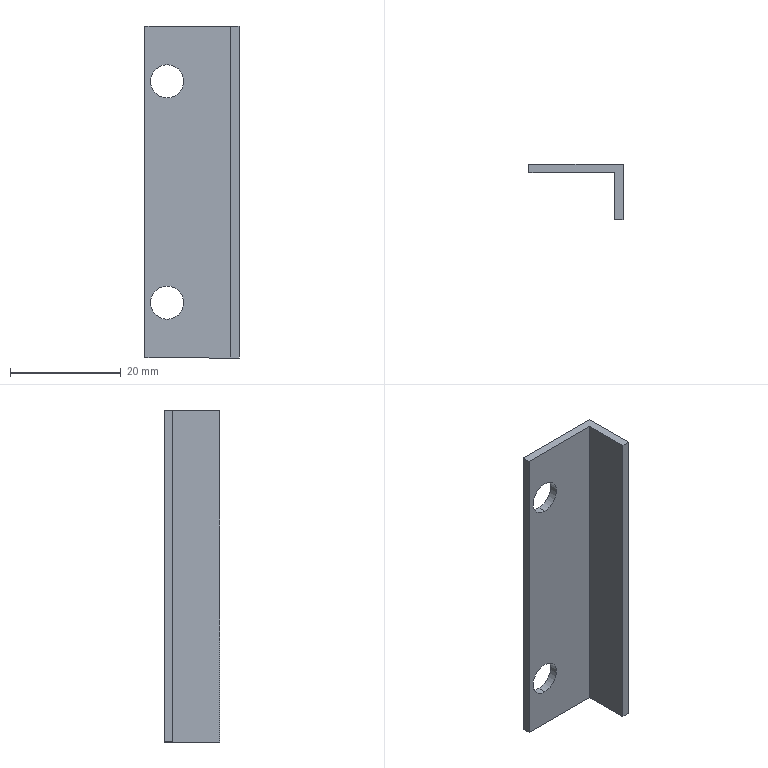Component | SolidWorks | RubberPlateBaffle-2 | 1 solid | 12 faces | box 17 x 10 x 60 mm | volume 2210 mm3 | plane 8 | cylinder 4 | commonest cylinder face diameters 6 x4
build123d program:
from build123d import *

# Parameters (mm, degrees)
SKETCH1_W                    = 60
SKETCH1_H                    = 17
BOSS_EXTRUDE1_DEPTH          = 10
SKETCH2_W                    = 8.5
SKETCH2_H                    = 15.5
CUT_EXTRUDE1_DEPTH           = 64.159
F_6_0_6_DIAMETER_HOLE1_D     = 6
F_6_0_6_DIAMETER_HOLE1_DEPTH = 10


with BuildPart() as part:
    # Sketch1 → Boss-Extrude1 (new body)
    with BuildSketch(Plane(origin=(10, 0, 0), x_dir=(0, 0, -1), z_dir=(1, 0, 0))):
        with Locations((0, 8.5)):
            Rectangle(SKETCH1_W, SKETCH1_H)
    extrude(amount=-BOSS_EXTRUDE1_DEPTH)

    # Sketch2 → Cut-Extrude1 (cut, through all)
    with BuildSketch(Plane.XY.offset(30)):
        with Locations((5.75, 9.25)):
            Rectangle(SKETCH2_W, SKETCH2_H)
    extrude(amount=-CUT_EXTRUDE1_DEPTH, mode=Mode.SUBTRACT)

    # 6.0 _6_ Diameter Hole1
    with Locations(Plane.ZY):
        with Locations((20, 13), (-20, 13)):
            Hole(F_6_0_6_DIAMETER_HOLE1_D / 2, depth=F_6_0_6_DIAMETER_HOLE1_DEPTH)


solid = part.part

# Placed as in the assembly
solid = solid.moved(Location((-382.5, 434.25, -73.487), (180, 0, 90)))
STEP:
#1=COLOUR_RGB('',0.7922,0.8196,0.9333);
#2=FILL_AREA_STYLE_COLOUR('',#1);
#3=FILL_AREA_STYLE('',(#2));
#4=SURFACE_STYLE_FILL_AREA(#3);
#5=SURFACE_SIDE_STYLE('',(#4));
#6=SURFACE_STYLE_USAGE(.BOTH.,#5);
#7=PRESENTATION_STYLE_ASSIGNMENT((#6));
#8=CARTESIAN_POINT('',(-15.571,17.037,-3.562));
#9=VERTEX_POINT('',#8);
#10=CARTESIAN_POINT('',(-15.571,17.037,-3.799));
#11=VERTEX_POINT('',#10);
#12=CARTESIAN_POINT('',(-15.571,17.037,-3.681));
#13=DIRECTION('',(0.,1.,-0.));
#14=DIRECTION('',(1.,0.,0.));
#15=AXIS2_PLACEMENT_3D('',#12,#13,#14);
#16=CIRCLE('',#15,0.1181);
#17=EDGE_CURVE('',#9,#11,#16,.T.);
#18=ORIENTED_EDGE('',*,*,#17,.F.);
#19=CARTESIAN_POINT('',(-15.571,17.096,-3.562));
#20=VERTEX_POINT('',#19);
#21=CARTESIAN_POINT('',(-15.571,17.096,-3.562));
#22=DIRECTION('',(0.,1.,-0.));
#23=VECTOR('',#22,39.37);
#24=LINE('',#21,#23);
#25=EDGE_CURVE('',#9,#20,#24,.T.);
#26=ORIENTED_EDGE('',*,*,#25,.T.);
#27=CARTESIAN_POINT('',(-15.571,17.096,-3.799));
#28=VERTEX_POINT('',#27);
#29=CARTESIAN_POINT('',(-15.571,17.096,-3.681));
#30=DIRECTION('',(0.,1.,-0.));
#31=DIRECTION('',(0.,0.,-1.));
#32=AXIS2_PLACEMENT_3D('',#29,#30,#31);
#33=CIRCLE('',#32,0.1181);
#34=EDGE_CURVE('',#20,#28,#33,.T.);
#35=ORIENTED_EDGE('',*,*,#34,.T.);
#36=CARTESIAN_POINT('',(-15.571,17.096,-3.799));
#37=DIRECTION('',(0.,1.,-0.));
#38=VECTOR('',#37,39.37);
#39=LINE('',#36,#38);
#40=EDGE_CURVE('',#11,#28,#39,.T.);
#41=ORIENTED_EDGE('',*,*,#40,.F.);
#42=EDGE_LOOP('',(#18,#26,#35,#41));
#43=FACE_OUTER_BOUND('',#42,.T.);
#44=CARTESIAN_POINT('',(-15.571,17.096,-3.681));
#45=DIRECTION('',(0.,1.,-0.));
#46=DIRECTION('',(0.,0.,-1.));
#47=AXIS2_PLACEMENT_3D('',#44,#45,#46);
#48=CYLINDRICAL_SURFACE('',#47,0.1181);
#49=ADVANCED_FACE('',(#43),#48,.F.);
#50=CARTESIAN_POINT('',(-15.571,17.037,-1.988));
#51=VERTEX_POINT('',#50);
#52=CARTESIAN_POINT('',(-15.571,17.037,-2.224));
#53=VERTEX_POINT('',#52);
#54=CARTESIAN_POINT('',(-15.571,17.037,-2.106));
#55=DIRECTION('',(0.,1.,-0.));
#56=DIRECTION('',(1.,0.,0.));
#57=AXIS2_PLACEMENT_3D('',#54,#55,#56);
#58=CIRCLE('',#57,0.1181);
#59=EDGE_CURVE('',#51,#53,#58,.T.);
#60=ORIENTED_EDGE('',*,*,#59,.F.);
#61=CARTESIAN_POINT('',(-15.571,17.096,-1.988));
#62=VERTEX_POINT('',#61);
#63=CARTESIAN_POINT('',(-15.571,17.096,-1.988));
#64=DIRECTION('',(0.,1.,-0.));
#65=VECTOR('',#64,39.37);
#66=LINE('',#63,#65);
#67=EDGE_CURVE('',#51,#62,#66,.T.);
#68=ORIENTED_EDGE('',*,*,#67,.T.);
#69=CARTESIAN_POINT('',(-15.571,17.096,-2.224));
#70=VERTEX_POINT('',#69);
#71=CARTESIAN_POINT('',(-15.571,17.096,-2.106));
#72=DIRECTION('',(0.,1.,-0.));
#73=DIRECTION('',(0.,0.,-1.));
#74=AXIS2_PLACEMENT_3D('',#71,#72,#73);
#75=CIRCLE('',#74,0.1181);
#76=EDGE_CURVE('',#62,#70,#75,.T.);
#77=ORIENTED_EDGE('',*,*,#76,.T.);
#78=CARTESIAN_POINT('',(-15.571,17.096,-2.224));
#79=DIRECTION('',(0.,1.,-0.));
#80=VECTOR('',#79,39.37);
#81=LINE('',#78,#80);
#82=EDGE_CURVE('',#53,#70,#81,.T.);
#83=ORIENTED_EDGE('',*,*,#82,.F.);
#84=EDGE_LOOP('',(#60,#68,#77,#83));
#85=FACE_OUTER_BOUND('',#84,.T.);
#86=CARTESIAN_POINT('',(-15.571,17.096,-2.106));
#87=DIRECTION('',(0.,1.,-0.));
#88=DIRECTION('',(0.,0.,-1.));
#89=AXIS2_PLACEMENT_3D('',#86,#87,#88);
#90=CYLINDRICAL_SURFACE('',#89,0.1181);
#91=ADVANCED_FACE('',(#85),#90,.F.);
#92=CARTESIAN_POINT('',(-15.728,17.037,-1.712));
#93=VERTEX_POINT('',#92);
#94=CARTESIAN_POINT('',(-15.728,17.037,-4.074));
#95=VERTEX_POINT('',#94);
#96=CARTESIAN_POINT('',(-15.728,17.037,-1.712));
#97=DIRECTION('',(-0.,-0.,-1.));
#98=VECTOR('',#97,39.37);
#99=LINE('',#96,#98);
#100=EDGE_CURVE('',#93,#95,#99,.T.);
#101=ORIENTED_EDGE('',*,*,#100,.F.);
#102=CARTESIAN_POINT('',(-15.728,17.096,-1.712));
#103=VERTEX_POINT('',#102);
#104=CARTESIAN_POINT('',(-15.728,17.096,-1.712));
#105=DIRECTION('',(-0.,-1.,0.));
#106=VECTOR('',#105,39.37);
#107=LINE('',#104,#106);
#108=EDGE_CURVE('',#103,#93,#107,.T.);
#109=ORIENTED_EDGE('',*,*,#108,.F.);
#110=CARTESIAN_POINT('',(-15.728,17.096,-4.074));
#111=VERTEX_POINT('',#110);
#112=CARTESIAN_POINT('',(-15.728,17.096,-1.712));
#113=DIRECTION('',(-0.,-0.,-1.));
#114=VECTOR('',#113,39.37);
#115=LINE('',#112,#114);
#116=EDGE_CURVE('',#103,#111,#115,.T.);
#117=ORIENTED_EDGE('',*,*,#116,.T.);
#118=CARTESIAN_POINT('',(-15.728,17.096,-4.074));
#119=DIRECTION('',(-0.,-1.,0.));
#120=VECTOR('',#119,39.37);
#121=LINE('',#118,#120);
#122=EDGE_CURVE('',#111,#95,#121,.T.);
#123=ORIENTED_EDGE('',*,*,#122,.T.);
#124=EDGE_LOOP('',(#101,#109,#117,#123));
#125=FACE_OUTER_BOUND('',#124,.T.);
#126=CARTESIAN_POINT('',(-15.728,17.096,-1.712));
#127=DIRECTION('',(-1.,0.,0.));
#128=DIRECTION('',(-0.,-0.,-1.));
#129=AXIS2_PLACEMENT_3D('',#126,#127,#128);
#130=PLANE('',#129);
#131=ADVANCED_FACE('',(#125),#130,.T.);
#132=CARTESIAN_POINT('',(-15.118,17.037,-1.712));
#133=VERTEX_POINT('',#132);
#134=CARTESIAN_POINT('',(-15.728,17.037,-1.712));
#135=DIRECTION('',(1.,-0.,-0.));
#136=VECTOR('',#135,39.37);
#137=LINE('',#134,#136);
#138=EDGE_CURVE('',#93,#133,#137,.T.);
#139=ORIENTED_EDGE('',*,*,#138,.T.);
#140=CARTESIAN_POINT('',(-15.118,16.703,-1.712));
#141=VERTEX_POINT('',#140);
#142=CARTESIAN_POINT('',(-15.118,17.037,-1.712));
#143=DIRECTION('',(-0.,-1.,0.));
#144=VECTOR('',#143,39.37);
#145=LINE('',#142,#144);
#146=EDGE_CURVE('',#133,#141,#145,.T.);
#147=ORIENTED_EDGE('',*,*,#146,.T.);
#148=CARTESIAN_POINT('',(-15.059,16.703,-1.712));
#149=VERTEX_POINT('',#148);
#150=CARTESIAN_POINT('',(-15.059,16.703,-1.712));
#151=DIRECTION('',(-1.,0.,0.));
#152=VECTOR('',#151,39.37);
#153=LINE('',#150,#152);
#154=EDGE_CURVE('',#149,#141,#153,.T.);
#155=ORIENTED_EDGE('',*,*,#154,.F.);
#156=CARTESIAN_POINT('',(-15.059,17.096,-1.712));
#157=VERTEX_POINT('',#156);
#158=CARTESIAN_POINT('',(-15.059,17.096,-1.712));
#159=DIRECTION('',(-0.,-1.,0.));
#160=VECTOR('',#159,39.37);
#161=LINE('',#158,#160);
#162=EDGE_CURVE('',#157,#149,#161,.T.);
#163=ORIENTED_EDGE('',*,*,#162,.F.);
#164=CARTESIAN_POINT('',(-15.059,17.096,-1.712));
#165=DIRECTION('',(-1.,0.,0.));
#166=VECTOR('',#165,39.37);
#167=LINE('',#164,#166);
#168=EDGE_CURVE('',#157,#103,#167,.T.);
#169=ORIENTED_EDGE('',*,*,#168,.T.);
#170=ORIENTED_EDGE('',*,*,#108,.T.);
#171=EDGE_LOOP('',(#139,#147,#155,#163,#169,#170));
#172=FACE_OUTER_BOUND('',#171,.T.);
#173=CARTESIAN_POINT('',(-15.059,17.096,-1.712));
#174=DIRECTION('',(0.,0.,1.));
#175=DIRECTION('',(0.,1.,-0.));
#176=AXIS2_PLACEMENT_3D('',#173,#174,#175);
#177=PLANE('',#176);
#178=ADVANCED_FACE('',(#172),#177,.T.);
#179=CARTESIAN_POINT('',(-15.059,16.703,-4.074));
#180=VERTEX_POINT('',#179);
#181=CARTESIAN_POINT('',(-15.059,16.703,-4.074));
#182=DIRECTION('',(0.,0.,1.));
#183=VECTOR('',#182,39.37);
#184=LINE('',#181,#183);
#185=EDGE_CURVE('',#180,#149,#184,.T.);
#186=ORIENTED_EDGE('',*,*,#185,.F.);
#187=CARTESIAN_POINT('',(-15.059,17.096,-4.074));
#188=VERTEX_POINT('',#187);
#189=CARTESIAN_POINT('',(-15.059,17.096,-4.074));
#190=DIRECTION('',(-0.,-1.,0.));
#191=VECTOR('',#190,39.37);
#192=LINE('',#189,#191);
#193=EDGE_CURVE('',#188,#180,#192,.T.);
#194=ORIENTED_EDGE('',*,*,#193,.F.);
#195=CARTESIAN_POINT('',(-15.059,17.096,-4.074));
#196=DIRECTION('',(0.,0.,1.));
#197=VECTOR('',#196,39.37);
#198=LINE('',#195,#197);
#199=EDGE_CURVE('',#188,#157,#198,.T.);
#200=ORIENTED_EDGE('',*,*,#199,.T.);
#201=ORIENTED_EDGE('',*,*,#162,.T.);
#202=EDGE_LOOP('',(#186,#194,#200,#201));
#203=FACE_OUTER_BOUND('',#202,.T.);
#204=CARTESIAN_POINT('',(-15.059,17.096,-4.074));
#205=DIRECTION('',(1.,-0.,-0.));
#206=DIRECTION('',(0.,0.,1.));
#207=AXIS2_PLACEMENT_3D('',#204,#205,#206);
#208=PLANE('',#207);
#209=ADVANCED_FACE('',(#203),#208,.T.);
#210=CARTESIAN_POINT('',(-15.118,17.037,-4.074));
#211=VERTEX_POINT('',#210);
#212=CARTESIAN_POINT('',(-15.728,17.037,-4.074));
#213=DIRECTION('',(1.,-0.,-0.));
#214=VECTOR('',#213,39.37);
#215=LINE('',#212,#214);
#216=EDGE_CURVE('',#95,#211,#215,.T.);
#217=ORIENTED_EDGE('',*,*,#216,.F.);
#218=ORIENTED_EDGE('',*,*,#122,.F.);
#219=CARTESIAN_POINT('',(-15.728,17.096,-4.074));
#220=DIRECTION('',(1.,-0.,-0.));
#221=VECTOR('',#220,39.37);
#222=LINE('',#219,#221);
#223=EDGE_CURVE('',#111,#188,#222,.T.);
#224=ORIENTED_EDGE('',*,*,#223,.T.);
#225=ORIENTED_EDGE('',*,*,#193,.T.);
#226=CARTESIAN_POINT('',(-15.118,16.703,-4.074));
#227=VERTEX_POINT('',#226);
#228=CARTESIAN_POINT('',(-15.728,16.703,-4.074));
#229=DIRECTION('',(1.,-0.,-0.));
#230=VECTOR('',#229,39.37);
#231=LINE('',#228,#230);
#232=EDGE_CURVE('',#227,#180,#231,.T.);
#233=ORIENTED_EDGE('',*,*,#232,.F.);
#234=CARTESIAN_POINT('',(-15.118,17.037,-4.074));
#235=DIRECTION('',(-0.,-1.,0.));
#236=VECTOR('',#235,39.37);
#237=LINE('',#234,#236);
#238=EDGE_CURVE('',#211,#227,#237,.T.);
#239=ORIENTED_EDGE('',*,*,#238,.F.);
#240=EDGE_LOOP('',(#217,#218,#224,#225,#233,#239));
#241=FACE_OUTER_BOUND('',#240,.T.);
#242=CARTESIAN_POINT('',(-15.728,17.096,-4.074));
#243=DIRECTION('',(-0.,-0.,-1.));
#244=DIRECTION('',(-0.,-1.,0.));
#245=AXIS2_PLACEMENT_3D('',#242,#243,#244);
#246=PLANE('',#245);
#247=ADVANCED_FACE('',(#241),#246,.T.);
#248=CARTESIAN_POINT('',(-15.571,17.096,-3.681));
#249=DIRECTION('',(0.,1.,-0.));
#250=DIRECTION('',(0.,0.,-1.));
#251=AXIS2_PLACEMENT_3D('',#248,#249,#250);
#252=CIRCLE('',#251,0.1181);
#253=EDGE_CURVE('',#28,#20,#252,.T.);
#254=ORIENTED_EDGE('',*,*,#253,.F.);
#255=ORIENTED_EDGE('',*,*,#34,.F.);
#256=EDGE_LOOP('',(#254,#255));
#257=FACE_BOUND('',#256,.T.);
#258=CARTESIAN_POINT('',(-15.571,17.096,-2.106));
#259=DIRECTION('',(0.,1.,-0.));
#260=DIRECTION('',(0.,0.,-1.));
#261=AXIS2_PLACEMENT_3D('',#258,#259,#260);
#262=CIRCLE('',#261,0.1181);
#263=EDGE_CURVE('',#70,#62,#262,.T.);
#264=ORIENTED_EDGE('',*,*,#263,.F.);
#265=ORIENTED_EDGE('',*,*,#76,.F.);
#266=EDGE_LOOP('',(#264,#265));
#267=FACE_BOUND('',#266,.T.);
#268=ORIENTED_EDGE('',*,*,#116,.F.);
#269=ORIENTED_EDGE('',*,*,#168,.F.);
#270=ORIENTED_EDGE('',*,*,#199,.F.);
#271=ORIENTED_EDGE('',*,*,#223,.F.);
#272=EDGE_LOOP('',(#268,#269,#270,#271));
#273=FACE_OUTER_BOUND('',#272,.T.);
#274=CARTESIAN_POINT('',(-15.059,17.096,-2.893));
#275=DIRECTION('',(-0.,-1.,0.));
#276=DIRECTION('',(0.,0.,1.));
#277=AXIS2_PLACEMENT_3D('',#274,#275,#276);
#278=PLANE('',#277);
#279=ADVANCED_FACE('',(#257,#267,#273),#278,.F.);
#280=CARTESIAN_POINT('',(-15.118,16.703,-1.712));
#281=DIRECTION('',(-0.,-0.,-1.));
#282=VECTOR('',#281,39.37);
#283=LINE('',#280,#282);
#284=EDGE_CURVE('',#141,#227,#283,.T.);
#285=ORIENTED_EDGE('',*,*,#284,.T.);
#286=ORIENTED_EDGE('',*,*,#232,.T.);
#287=ORIENTED_EDGE('',*,*,#185,.T.);
#288=ORIENTED_EDGE('',*,*,#154,.T.);
#289=EDGE_LOOP('',(#285,#286,#287,#288));
#290=FACE_OUTER_BOUND('',#289,.T.);
#291=CARTESIAN_POINT('',(-15.059,16.703,-2.893));
#292=DIRECTION('',(-0.,-1.,0.));
#293=DIRECTION('',(0.,0.,1.));
#294=AXIS2_PLACEMENT_3D('',#291,#292,#293);
#295=PLANE('',#294);
#296=ADVANCED_FACE('',(#290),#295,.T.);
#297=CARTESIAN_POINT('',(-15.571,17.037,-3.681));
#298=DIRECTION('',(0.,1.,-0.));
#299=DIRECTION('',(1.,0.,0.));
#300=AXIS2_PLACEMENT_3D('',#297,#298,#299);
#301=CIRCLE('',#300,0.1181);
#302=EDGE_CURVE('',#11,#9,#301,.T.);
#303=ORIENTED_EDGE('',*,*,#302,.T.);
#304=ORIENTED_EDGE('',*,*,#17,.T.);
#305=EDGE_LOOP('',(#303,#304));
#306=FACE_BOUND('',#305,.T.);
#307=CARTESIAN_POINT('',(-15.571,17.037,-2.106));
#308=DIRECTION('',(0.,1.,-0.));
#309=DIRECTION('',(1.,0.,0.));
#310=AXIS2_PLACEMENT_3D('',#307,#308,#309);
#311=CIRCLE('',#310,0.1181);
#312=EDGE_CURVE('',#53,#51,#311,.T.);
#313=ORIENTED_EDGE('',*,*,#312,.T.);
#314=ORIENTED_EDGE('',*,*,#59,.T.);
#315=EDGE_LOOP('',(#313,#314));
#316=FACE_BOUND('',#315,.T.);
#317=ORIENTED_EDGE('',*,*,#216,.T.);
#318=CARTESIAN_POINT('',(-15.118,17.037,-1.712));
#319=DIRECTION('',(-0.,-0.,-1.));
#320=VECTOR('',#319,39.37);
#321=LINE('',#318,#320);
#322=EDGE_CURVE('',#133,#211,#321,.T.);
#323=ORIENTED_EDGE('',*,*,#322,.F.);
#324=ORIENTED_EDGE('',*,*,#138,.F.);
#325=ORIENTED_EDGE('',*,*,#100,.T.);
#326=EDGE_LOOP('',(#317,#323,#324,#325));
#327=FACE_OUTER_BOUND('',#326,.T.);
#328=CARTESIAN_POINT('',(-15.728,17.037,-1.712));
#329=DIRECTION('',(0.,1.,-0.));
#330=DIRECTION('',(1.,-0.,-0.));
#331=AXIS2_PLACEMENT_3D('',#328,#329,#330);
#332=PLANE('',#331);
#333=ADVANCED_FACE('',(#306,#316,#327),#332,.F.);
#334=ORIENTED_EDGE('',*,*,#238,.T.);
#335=ORIENTED_EDGE('',*,*,#284,.F.);
#336=ORIENTED_EDGE('',*,*,#146,.F.);
#337=ORIENTED_EDGE('',*,*,#322,.T.);
#338=EDGE_LOOP('',(#334,#335,#336,#337));
#339=FACE_OUTER_BOUND('',#338,.T.);
#340=CARTESIAN_POINT('',(-15.118,17.037,-1.712));
#341=DIRECTION('',(1.,-0.,-0.));
#342=DIRECTION('',(0.,0.,1.));
#343=AXIS2_PLACEMENT_3D('',#340,#341,#342);
#344=PLANE('',#343);
#345=ADVANCED_FACE('',(#339),#344,.F.);
#346=ORIENTED_EDGE('',*,*,#67,.F.);
#347=ORIENTED_EDGE('',*,*,#312,.F.);
#348=ORIENTED_EDGE('',*,*,#82,.T.);
#349=ORIENTED_EDGE('',*,*,#263,.T.);
#350=EDGE_LOOP('',(#346,#347,#348,#349));
#351=FACE_OUTER_BOUND('',#350,.T.);
#352=CARTESIAN_POINT('',(-15.571,17.096,-2.106));
#353=DIRECTION('',(0.,1.,-0.));
#354=DIRECTION('',(0.,0.,-1.));
#355=AXIS2_PLACEMENT_3D('',#352,#353,#354);
#356=CYLINDRICAL_SURFACE('',#355,0.1181);
#357=ADVANCED_FACE('',(#351),#356,.F.);
#358=ORIENTED_EDGE('',*,*,#25,.F.);
#359=ORIENTED_EDGE('',*,*,#302,.F.);
#360=ORIENTED_EDGE('',*,*,#40,.T.);
#361=ORIENTED_EDGE('',*,*,#253,.T.);
#362=EDGE_LOOP('',(#358,#359,#360,#361));
#363=FACE_OUTER_BOUND('',#362,.T.);
#364=CARTESIAN_POINT('',(-15.571,17.096,-3.681));
#365=DIRECTION('',(0.,1.,-0.));
#366=DIRECTION('',(0.,0.,-1.));
#367=AXIS2_PLACEMENT_3D('',#364,#365,#366);
#368=CYLINDRICAL_SURFACE('',#367,0.1181);
#369=ADVANCED_FACE('',(#363),#368,.F.);
#370=CLOSED_SHELL('',(#49,#91,#131,#178,#209,#247,#279,#296,#333,#345,#357,#369));
#371=MANIFOLD_SOLID_BREP('',#370);
#372=STYLED_ITEM('',(#7),#371);
#373=(LENGTH_UNIT()NAMED_UNIT(*)SI_UNIT($,.METRE.));
#374=LENGTH_MEASURE_WITH_UNIT(LENGTH_MEASURE(0.0254),#373);
#375=DIMENSIONAL_EXPONENTS(1.,0.,0.,0.,0.,0.,0.);
#376=(CONVERSION_BASED_UNIT('',#374)LENGTH_UNIT()NAMED_UNIT(#375));
#377=UNCERTAINTY_MEASURE_WITH_UNIT(LENGTH_MEASURE(0.00001),#376,'','');
#378=(NAMED_UNIT(*)PLANE_ANGLE_UNIT()SI_UNIT($,.RADIAN.));
#379=(NAMED_UNIT(*)SI_UNIT($,.STERADIAN.)SOLID_ANGLE_UNIT());
#380=(GEOMETRIC_REPRESENTATION_CONTEXT(3)GLOBAL_UNCERTAINTY_ASSIGNED_CONTEXT((#377))GLOBAL_UNIT_ASSIGNED_CONTEXT((#376,#378,#379))REPRESENTATION_CONTEXT('',''));
#381=MECHANICAL_DESIGN_GEOMETRIC_PRESENTATION_REPRESENTATION('',(#372),#380);
#382=CARTESIAN_POINT('',(0.,0.,0.));
#383=DIRECTION('',(0.,0.,1.));
#384=DIRECTION('',(1.,0.,0.));
#385=AXIS2_PLACEMENT_3D('',#382,#383,#384);
#386=(LENGTH_UNIT()NAMED_UNIT(*)SI_UNIT($,.METRE.));
#387=LENGTH_MEASURE_WITH_UNIT(LENGTH_MEASURE(0.0254),#386);
#388=DIMENSIONAL_EXPONENTS(1.,0.,0.,0.,0.,0.,0.);
#389=(CONVERSION_BASED_UNIT('',#387)LENGTH_UNIT()NAMED_UNIT(#388));
#390=UNCERTAINTY_MEASURE_WITH_UNIT(LENGTH_MEASURE(0.00001),#389,'','');
#391=(NAMED_UNIT(*)PLANE_ANGLE_UNIT()SI_UNIT($,.RADIAN.));
#392=(NAMED_UNIT(*)SI_UNIT($,.STERADIAN.)SOLID_ANGLE_UNIT());
#393=(GEOMETRIC_REPRESENTATION_CONTEXT(3)GLOBAL_UNCERTAINTY_ASSIGNED_CONTEXT((#390))GLOBAL_UNIT_ASSIGNED_CONTEXT((#389,#391,#392))REPRESENTATION_CONTEXT('',''));
#394=ADVANCED_BREP_SHAPE_REPRESENTATION('',(#371,#385),#393);
#395=PRESENTATION_LAYER_ASSIGNMENT('','',(#372));